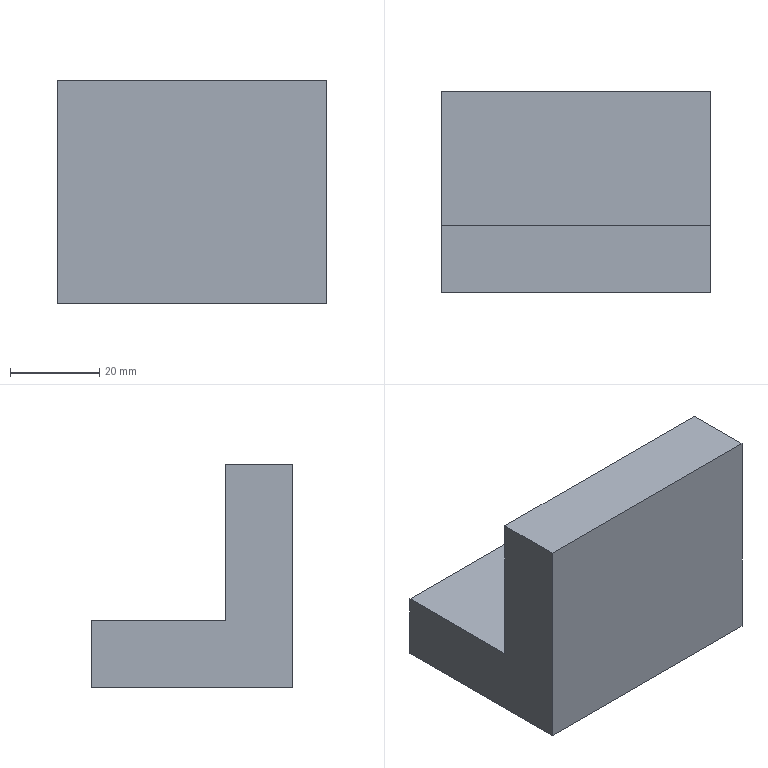Component | SolidWorks | Part10-2 | 1 solid | 8 faces | box 60 x 45 x 50 mm | volume 72000 mm3 | plane 8
build123d program:
from build123d import *

# Parameters (mm, degrees)
BOSS_EXTRUDE1_DEPTH = 30


with BuildPart() as part:
    # Sketch1 → Boss-Extrude1 (new, symmetric)
    with BuildSketch(Plane(origin=(0, 0, 0), x_dir=(0, 0, -1), z_dir=(1, 0, 0))):
        Polygon((0, 0), (0, 45), (-15, 45), (-15, 15), (-50, 15), (-50, 0), align=None)
    extrude(amount=BOSS_EXTRUDE1_DEPTH, both=True)


solid = part.part

# Placed as in the assembly
solid = solid.moved(Location((-87.007, -466, -410), (0, 0, 0)))
STEP:
#1=COLOUR_RGB('',0.7922,0.8196,0.9333);
#2=FILL_AREA_STYLE_COLOUR('',#1);
#3=FILL_AREA_STYLE('',(#2));
#4=SURFACE_STYLE_FILL_AREA(#3);
#5=SURFACE_SIDE_STYLE('',(#4));
#6=SURFACE_STYLE_USAGE(.BOTH.,#5);
#7=PRESENTATION_STYLE_ASSIGNMENT((#6));
#8=CARTESIAN_POINT('',(-4.607,-18.346,-14.173));
#9=VERTEX_POINT('',#8);
#10=CARTESIAN_POINT('',(-4.607,-18.346,-16.142));
#11=VERTEX_POINT('',#10);
#12=CARTESIAN_POINT('',(-4.607,-18.346,-14.173));
#13=DIRECTION('',(0.,0.,-1.));
#14=VECTOR('',#13,39.37);
#15=LINE('',#12,#14);
#16=EDGE_CURVE('',#9,#11,#15,.T.);
#17=ORIENTED_EDGE('',*,*,#16,.T.);
#18=CARTESIAN_POINT('',(-2.244,-18.346,-16.142));
#19=VERTEX_POINT('',#18);
#20=CARTESIAN_POINT('',(-2.244,-18.346,-16.142));
#21=DIRECTION('',(-1.,0.,0.));
#22=VECTOR('',#21,39.37);
#23=LINE('',#20,#22);
#24=EDGE_CURVE('',#19,#11,#23,.T.);
#25=ORIENTED_EDGE('',*,*,#24,.F.);
#26=CARTESIAN_POINT('',(-2.244,-18.346,-14.173));
#27=VERTEX_POINT('',#26);
#28=CARTESIAN_POINT('',(-2.244,-18.346,-14.173));
#29=DIRECTION('',(0.,0.,-1.));
#30=VECTOR('',#29,39.37);
#31=LINE('',#28,#30);
#32=EDGE_CURVE('',#27,#19,#31,.T.);
#33=ORIENTED_EDGE('',*,*,#32,.F.);
#34=CARTESIAN_POINT('',(-2.244,-18.346,-14.173));
#35=DIRECTION('',(-1.,0.,0.));
#36=VECTOR('',#35,39.37);
#37=LINE('',#34,#36);
#38=EDGE_CURVE('',#27,#9,#37,.T.);
#39=ORIENTED_EDGE('',*,*,#38,.T.);
#40=EDGE_LOOP('',(#17,#25,#33,#39));
#41=FACE_OUTER_BOUND('',#40,.T.);
#42=CARTESIAN_POINT('',(-2.244,-18.346,-14.173));
#43=DIRECTION('',(0.,1.,0.));
#44=DIRECTION('',(0.,0.,1.));
#45=AXIS2_PLACEMENT_3D('',#42,#43,#44);
#46=PLANE('',#45);
#47=ADVANCED_FACE('',(#41),#46,.F.);
#48=CARTESIAN_POINT('',(-4.607,-16.575,-16.142));
#49=VERTEX_POINT('',#48);
#50=CARTESIAN_POINT('',(-4.607,-18.346,-16.142));
#51=DIRECTION('',(0.,1.,0.));
#52=VECTOR('',#51,39.37);
#53=LINE('',#50,#52);
#54=EDGE_CURVE('',#11,#49,#53,.T.);
#55=ORIENTED_EDGE('',*,*,#54,.T.);
#56=CARTESIAN_POINT('',(-2.244,-16.575,-16.142));
#57=VERTEX_POINT('',#56);
#58=CARTESIAN_POINT('',(-2.244,-16.575,-16.142));
#59=DIRECTION('',(-1.,0.,0.));
#60=VECTOR('',#59,39.37);
#61=LINE('',#58,#60);
#62=EDGE_CURVE('',#57,#49,#61,.T.);
#63=ORIENTED_EDGE('',*,*,#62,.F.);
#64=CARTESIAN_POINT('',(-2.244,-18.346,-16.142));
#65=DIRECTION('',(0.,1.,0.));
#66=VECTOR('',#65,39.37);
#67=LINE('',#64,#66);
#68=EDGE_CURVE('',#19,#57,#67,.T.);
#69=ORIENTED_EDGE('',*,*,#68,.F.);
#70=ORIENTED_EDGE('',*,*,#24,.T.);
#71=EDGE_LOOP('',(#55,#63,#69,#70));
#72=FACE_OUTER_BOUND('',#71,.T.);
#73=CARTESIAN_POINT('',(-2.244,-18.346,-16.142));
#74=DIRECTION('',(0.,0.,1.));
#75=DIRECTION('',(1.,0.,0.));
#76=AXIS2_PLACEMENT_3D('',#73,#74,#75);
#77=PLANE('',#76);
#78=ADVANCED_FACE('',(#72),#77,.F.);
#79=CARTESIAN_POINT('',(-4.607,-16.575,-15.551));
#80=VERTEX_POINT('',#79);
#81=CARTESIAN_POINT('',(-4.607,-16.575,-16.142));
#82=DIRECTION('',(0.,0.,1.));
#83=VECTOR('',#82,39.37);
#84=LINE('',#81,#83);
#85=EDGE_CURVE('',#49,#80,#84,.T.);
#86=ORIENTED_EDGE('',*,*,#85,.T.);
#87=CARTESIAN_POINT('',(-2.244,-16.575,-15.551));
#88=VERTEX_POINT('',#87);
#89=CARTESIAN_POINT('',(-2.244,-16.575,-15.551));
#90=DIRECTION('',(-1.,0.,0.));
#91=VECTOR('',#90,39.37);
#92=LINE('',#89,#91);
#93=EDGE_CURVE('',#88,#80,#92,.T.);
#94=ORIENTED_EDGE('',*,*,#93,.F.);
#95=CARTESIAN_POINT('',(-2.244,-16.575,-16.142));
#96=DIRECTION('',(0.,0.,1.));
#97=VECTOR('',#96,39.37);
#98=LINE('',#95,#97);
#99=EDGE_CURVE('',#57,#88,#98,.T.);
#100=ORIENTED_EDGE('',*,*,#99,.F.);
#101=ORIENTED_EDGE('',*,*,#62,.T.);
#102=EDGE_LOOP('',(#86,#94,#100,#101));
#103=FACE_OUTER_BOUND('',#102,.T.);
#104=CARTESIAN_POINT('',(-2.244,-16.575,-16.142));
#105=DIRECTION('',(0.,-1.,0.));
#106=DIRECTION('',(0.,0.,-1.));
#107=AXIS2_PLACEMENT_3D('',#104,#105,#106);
#108=PLANE('',#107);
#109=ADVANCED_FACE('',(#103),#108,.F.);
#110=CARTESIAN_POINT('',(-4.607,-17.756,-15.551));
#111=VERTEX_POINT('',#110);
#112=CARTESIAN_POINT('',(-4.607,-16.575,-15.551));
#113=DIRECTION('',(0.,-1.,-0.));
#114=VECTOR('',#113,39.37);
#115=LINE('',#112,#114);
#116=EDGE_CURVE('',#80,#111,#115,.T.);
#117=ORIENTED_EDGE('',*,*,#116,.T.);
#118=CARTESIAN_POINT('',(-2.244,-17.756,-15.551));
#119=VERTEX_POINT('',#118);
#120=CARTESIAN_POINT('',(-2.244,-17.756,-15.551));
#121=DIRECTION('',(-1.,0.,0.));
#122=VECTOR('',#121,39.37);
#123=LINE('',#120,#122);
#124=EDGE_CURVE('',#119,#111,#123,.T.);
#125=ORIENTED_EDGE('',*,*,#124,.F.);
#126=CARTESIAN_POINT('',(-2.244,-16.575,-15.551));
#127=DIRECTION('',(0.,-1.,-0.));
#128=VECTOR('',#127,39.37);
#129=LINE('',#126,#128);
#130=EDGE_CURVE('',#88,#119,#129,.T.);
#131=ORIENTED_EDGE('',*,*,#130,.F.);
#132=ORIENTED_EDGE('',*,*,#93,.T.);
#133=EDGE_LOOP('',(#117,#125,#131,#132));
#134=FACE_OUTER_BOUND('',#133,.T.);
#135=CARTESIAN_POINT('',(-2.244,-16.575,-15.551));
#136=DIRECTION('',(0.,0.,-1.));
#137=DIRECTION('',(0.,1.,0.));
#138=AXIS2_PLACEMENT_3D('',#135,#136,#137);
#139=PLANE('',#138);
#140=ADVANCED_FACE('',(#134),#139,.F.);
#141=CARTESIAN_POINT('',(-4.607,-17.756,-14.173));
#142=VERTEX_POINT('',#141);
#143=CARTESIAN_POINT('',(-4.607,-17.756,-15.551));
#144=DIRECTION('',(0.,-0.,1.));
#145=VECTOR('',#144,39.37);
#146=LINE('',#143,#145);
#147=EDGE_CURVE('',#111,#142,#146,.T.);
#148=ORIENTED_EDGE('',*,*,#147,.T.);
#149=CARTESIAN_POINT('',(-2.244,-17.756,-14.173));
#150=VERTEX_POINT('',#149);
#151=CARTESIAN_POINT('',(-2.244,-17.756,-14.173));
#152=DIRECTION('',(-1.,0.,0.));
#153=VECTOR('',#152,39.37);
#154=LINE('',#151,#153);
#155=EDGE_CURVE('',#150,#142,#154,.T.);
#156=ORIENTED_EDGE('',*,*,#155,.F.);
#157=CARTESIAN_POINT('',(-2.244,-17.756,-15.551));
#158=DIRECTION('',(0.,-0.,1.));
#159=VECTOR('',#158,39.37);
#160=LINE('',#157,#159);
#161=EDGE_CURVE('',#119,#150,#160,.T.);
#162=ORIENTED_EDGE('',*,*,#161,.F.);
#163=ORIENTED_EDGE('',*,*,#124,.T.);
#164=EDGE_LOOP('',(#148,#156,#162,#163));
#165=FACE_OUTER_BOUND('',#164,.T.);
#166=CARTESIAN_POINT('',(-2.244,-17.756,-15.551));
#167=DIRECTION('',(0.,-1.,-0.));
#168=DIRECTION('',(0.,0.,-1.));
#169=AXIS2_PLACEMENT_3D('',#166,#167,#168);
#170=PLANE('',#169);
#171=ADVANCED_FACE('',(#165),#170,.F.);
#172=CARTESIAN_POINT('',(-4.607,-17.756,-14.173));
#173=DIRECTION('',(0.,-1.,0.));
#174=VECTOR('',#173,39.37);
#175=LINE('',#172,#174);
#176=EDGE_CURVE('',#142,#9,#175,.T.);
#177=ORIENTED_EDGE('',*,*,#176,.T.);
#178=ORIENTED_EDGE('',*,*,#38,.F.);
#179=CARTESIAN_POINT('',(-2.244,-17.756,-14.173));
#180=DIRECTION('',(0.,-1.,0.));
#181=VECTOR('',#180,39.37);
#182=LINE('',#179,#181);
#183=EDGE_CURVE('',#150,#27,#182,.T.);
#184=ORIENTED_EDGE('',*,*,#183,.F.);
#185=ORIENTED_EDGE('',*,*,#155,.T.);
#186=EDGE_LOOP('',(#177,#178,#184,#185));
#187=FACE_OUTER_BOUND('',#186,.T.);
#188=CARTESIAN_POINT('',(-2.244,-17.756,-14.173));
#189=DIRECTION('',(0.,0.,-1.));
#190=DIRECTION('',(-1.,0.,0.));
#191=AXIS2_PLACEMENT_3D('',#188,#189,#190);
#192=PLANE('',#191);
#193=ADVANCED_FACE('',(#187),#192,.F.);
#194=ORIENTED_EDGE('',*,*,#32,.T.);
#195=ORIENTED_EDGE('',*,*,#68,.T.);
#196=ORIENTED_EDGE('',*,*,#99,.T.);
#197=ORIENTED_EDGE('',*,*,#130,.T.);
#198=ORIENTED_EDGE('',*,*,#161,.T.);
#199=ORIENTED_EDGE('',*,*,#183,.T.);
#200=EDGE_LOOP('',(#194,#195,#196,#197,#198,#199));
#201=FACE_OUTER_BOUND('',#200,.T.);
#202=CARTESIAN_POINT('',(-2.244,-18.346,-16.142));
#203=DIRECTION('',(1.,0.,0.));
#204=DIRECTION('',(0.,0.,-1.));
#205=AXIS2_PLACEMENT_3D('',#202,#203,#204);
#206=PLANE('',#205);
#207=ADVANCED_FACE('',(#201),#206,.T.);
#208=ORIENTED_EDGE('',*,*,#16,.F.);
#209=ORIENTED_EDGE('',*,*,#176,.F.);
#210=ORIENTED_EDGE('',*,*,#147,.F.);
#211=ORIENTED_EDGE('',*,*,#116,.F.);
#212=ORIENTED_EDGE('',*,*,#85,.F.);
#213=ORIENTED_EDGE('',*,*,#54,.F.);
#214=EDGE_LOOP('',(#208,#209,#210,#211,#212,#213));
#215=FACE_OUTER_BOUND('',#214,.T.);
#216=CARTESIAN_POINT('',(-4.607,-18.346,-16.142));
#217=DIRECTION('',(1.,0.,0.));
#218=DIRECTION('',(0.,0.,-1.));
#219=AXIS2_PLACEMENT_3D('',#216,#217,#218);
#220=PLANE('',#219);
#221=ADVANCED_FACE('',(#215),#220,.F.);
#222=CLOSED_SHELL('',(#47,#78,#109,#140,#171,#193,#207,#221));
#223=MANIFOLD_SOLID_BREP('',#222);
#224=STYLED_ITEM('',(#7),#223);
#225=(LENGTH_UNIT()NAMED_UNIT(*)SI_UNIT($,.METRE.));
#226=LENGTH_MEASURE_WITH_UNIT(LENGTH_MEASURE(0.0254),#225);
#227=DIMENSIONAL_EXPONENTS(1.,0.,0.,0.,0.,0.,0.);
#228=(CONVERSION_BASED_UNIT('',#226)LENGTH_UNIT()NAMED_UNIT(#227));
#229=UNCERTAINTY_MEASURE_WITH_UNIT(LENGTH_MEASURE(0.00001),#228,'','');
#230=(NAMED_UNIT(*)PLANE_ANGLE_UNIT()SI_UNIT($,.RADIAN.));
#231=(NAMED_UNIT(*)SI_UNIT($,.STERADIAN.)SOLID_ANGLE_UNIT());
#232=(GEOMETRIC_REPRESENTATION_CONTEXT(3)GLOBAL_UNCERTAINTY_ASSIGNED_CONTEXT((#229))GLOBAL_UNIT_ASSIGNED_CONTEXT((#228,#230,#231))REPRESENTATION_CONTEXT('',''));
#233=MECHANICAL_DESIGN_GEOMETRIC_PRESENTATION_REPRESENTATION('',(#224),#232);
#234=PRESENTATION_LAYER_ASSIGNMENT('','',(#224));
#235=CARTESIAN_POINT('',(0.,0.,0.));
#236=DIRECTION('',(0.,0.,1.));
#237=DIRECTION('',(1.,0.,0.));
#238=AXIS2_PLACEMENT_3D('',#235,#236,#237);
#239=(LENGTH_UNIT()NAMED_UNIT(*)SI_UNIT($,.METRE.));
#240=LENGTH_MEASURE_WITH_UNIT(LENGTH_MEASURE(0.0254),#239);
#241=DIMENSIONAL_EXPONENTS(1.,0.,0.,0.,0.,0.,0.);
#242=(CONVERSION_BASED_UNIT('',#240)LENGTH_UNIT()NAMED_UNIT(#241));
#243=UNCERTAINTY_MEASURE_WITH_UNIT(LENGTH_MEASURE(0.00001),#242,'','');
#244=(NAMED_UNIT(*)PLANE_ANGLE_UNIT()SI_UNIT($,.RADIAN.));
#245=(NAMED_UNIT(*)SI_UNIT($,.STERADIAN.)SOLID_ANGLE_UNIT());
#246=(GEOMETRIC_REPRESENTATION_CONTEXT(3)GLOBAL_UNCERTAINTY_ASSIGNED_CONTEXT((#243))GLOBAL_UNIT_ASSIGNED_CONTEXT((#242,#244,#245))REPRESENTATION_CONTEXT('',''));
#247=ADVANCED_BREP_SHAPE_REPRESENTATION('',(#223,#238),#246);